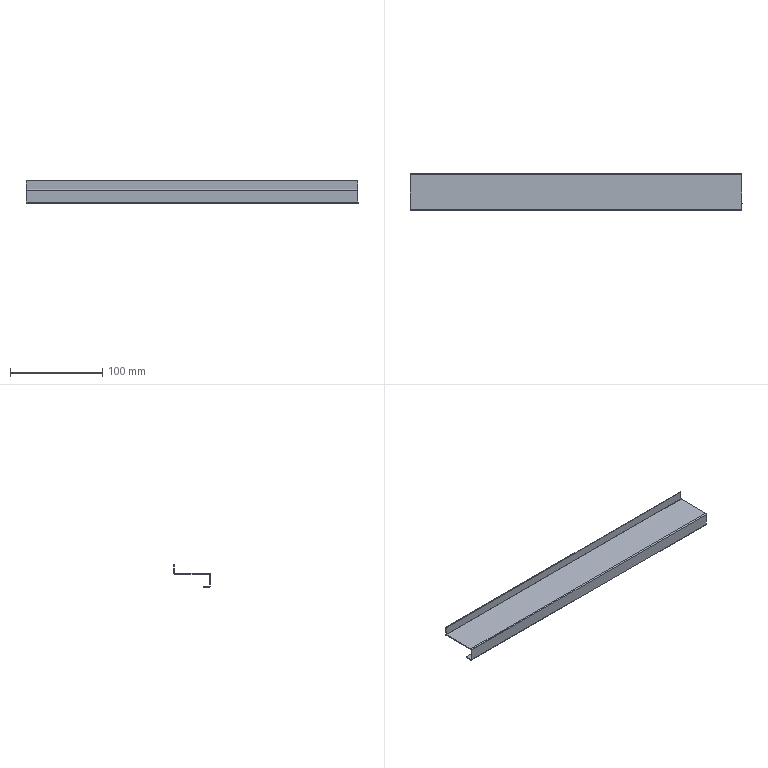Component | SolidWorks | MainBodyWeldment-1_UpperBeam-1 | 1 solid | 30 faces | box 360 x 40 x 24 mm | volume 24922 mm3 | plane 24 | cylinder 6 | commonest cylinder face diameters 0.2 x3 2.2 x3 | material SPCC
STEP:
#1=COLOUR_RGB('',0.7922,0.8196,0.9333);
#2=FILL_AREA_STYLE_COLOUR('',#1);
#3=FILL_AREA_STYLE('',(#2));
#4=SURFACE_STYLE_FILL_AREA(#3);
#5=SURFACE_SIDE_STYLE('',(#4));
#6=SURFACE_STYLE_USAGE(.BOTH.,#5);
#7=PRESENTATION_STYLE_ASSIGNMENT((#6));
#8=CARTESIAN_POINT('',(-7.236,13.105,9.799));
#9=VERTEX_POINT('',#8);
#10=CARTESIAN_POINT('',(-7.236,13.105,9.295));
#11=VERTEX_POINT('',#10);
#12=CARTESIAN_POINT('',(-7.236,13.105,9.843));
#13=DIRECTION('',(0.,0.,-1.));
#14=VECTOR('',#13,39.37);
#15=LINE('',#12,#14);
#16=EDGE_CURVE('',#9,#11,#15,.T.);
#17=ORIENTED_EDGE('',*,*,#16,.T.);
#18=CARTESIAN_POINT('',(-7.236,13.066,9.295));
#19=VERTEX_POINT('',#18);
#20=CARTESIAN_POINT('',(-7.236,13.105,9.295));
#21=DIRECTION('',(-0.,-1.,0.));
#22=VECTOR('',#21,39.37);
#23=LINE('',#20,#22);
#24=EDGE_CURVE('',#11,#19,#23,.T.);
#25=ORIENTED_EDGE('',*,*,#24,.T.);
#26=CARTESIAN_POINT('',(-7.236,13.066,9.799));
#27=VERTEX_POINT('',#26);
#28=CARTESIAN_POINT('',(-7.236,13.066,9.843));
#29=DIRECTION('',(0.,0.,-1.));
#30=VECTOR('',#29,39.37);
#31=LINE('',#28,#30);
#32=EDGE_CURVE('',#27,#19,#31,.T.);
#33=ORIENTED_EDGE('',*,*,#32,.F.);
#34=CARTESIAN_POINT('',(-7.236,13.066,9.799));
#35=DIRECTION('',(0.,1.,0.));
#36=VECTOR('',#35,39.37);
#37=LINE('',#34,#36);
#38=EDGE_CURVE('',#27,#9,#37,.T.);
#39=ORIENTED_EDGE('',*,*,#38,.T.);
#40=EDGE_LOOP('',(#17,#25,#33,#39));
#41=FACE_OUTER_BOUND('',#40,.T.);
#42=CARTESIAN_POINT('',(-7.236,13.109,9.803));
#43=DIRECTION('',(-1.,0.,0.));
#44=DIRECTION('',(0.,0.,1.));
#45=AXIS2_PLACEMENT_3D('',#42,#43,#44);
#46=PLANE('',#45);
#47=ADVANCED_FACE('',(#41),#46,.T.);
#48=CARTESIAN_POINT('',(6.938,13.066,9.295));
#49=VERTEX_POINT('',#48);
#50=CARTESIAN_POINT('',(-7.236,13.066,9.295));
#51=DIRECTION('',(1.,0.,0.));
#52=VECTOR('',#51,39.37);
#53=LINE('',#50,#52);
#54=EDGE_CURVE('',#19,#49,#53,.T.);
#55=ORIENTED_EDGE('',*,*,#54,.T.);
#56=CARTESIAN_POINT('',(6.938,13.066,9.799));
#57=VERTEX_POINT('',#56);
#58=CARTESIAN_POINT('',(6.938,13.066,9.843));
#59=DIRECTION('',(0.,0.,-1.));
#60=VECTOR('',#59,39.37);
#61=LINE('',#58,#60);
#62=EDGE_CURVE('',#57,#49,#61,.T.);
#63=ORIENTED_EDGE('',*,*,#62,.F.);
#64=CARTESIAN_POINT('',(6.938,13.066,9.799));
#65=DIRECTION('',(-1.,0.,0.));
#66=VECTOR('',#65,39.37);
#67=LINE('',#64,#66);
#68=EDGE_CURVE('',#57,#27,#67,.T.);
#69=ORIENTED_EDGE('',*,*,#68,.T.);
#70=ORIENTED_EDGE('',*,*,#32,.T.);
#71=EDGE_LOOP('',(#55,#63,#69,#70));
#72=FACE_OUTER_BOUND('',#71,.T.);
#73=CARTESIAN_POINT('',(6.938,13.066,9.843));
#74=DIRECTION('',(0.,1.,0.));
#75=DIRECTION('',(0.,0.,1.));
#76=AXIS2_PLACEMENT_3D('',#73,#74,#75);
#77=PLANE('',#76);
#78=ADVANCED_FACE('',(#72),#77,.F.);
#79=CARTESIAN_POINT('',(6.938,13.105,9.799));
#80=VERTEX_POINT('',#79);
#81=CARTESIAN_POINT('',(6.938,13.105,9.295));
#82=VERTEX_POINT('',#81);
#83=CARTESIAN_POINT('',(6.938,13.105,9.843));
#84=DIRECTION('',(0.,0.,-1.));
#85=VECTOR('',#84,39.37);
#86=LINE('',#83,#85);
#87=EDGE_CURVE('',#80,#82,#86,.T.);
#88=ORIENTED_EDGE('',*,*,#87,.T.);
#89=CARTESIAN_POINT('',(-7.236,13.105,9.295));
#90=DIRECTION('',(1.,0.,0.));
#91=VECTOR('',#90,39.37);
#92=LINE('',#89,#91);
#93=EDGE_CURVE('',#11,#82,#92,.T.);
#94=ORIENTED_EDGE('',*,*,#93,.F.);
#95=ORIENTED_EDGE('',*,*,#16,.F.);
#96=CARTESIAN_POINT('',(6.938,13.105,9.799));
#97=DIRECTION('',(-1.,0.,0.));
#98=VECTOR('',#97,39.37);
#99=LINE('',#96,#98);
#100=EDGE_CURVE('',#80,#9,#99,.T.);
#101=ORIENTED_EDGE('',*,*,#100,.F.);
#102=EDGE_LOOP('',(#88,#94,#95,#101));
#103=FACE_OUTER_BOUND('',#102,.T.);
#104=CARTESIAN_POINT('',(6.938,13.105,9.843));
#105=DIRECTION('',(0.,1.,0.));
#106=DIRECTION('',(0.,0.,1.));
#107=AXIS2_PLACEMENT_3D('',#104,#105,#106);
#108=PLANE('',#107);
#109=ADVANCED_FACE('',(#103),#108,.T.);
#110=CARTESIAN_POINT('',(6.938,13.109,9.843));
#111=VERTEX_POINT('',#110);
#112=CARTESIAN_POINT('',(6.938,13.109,9.803));
#113=VERTEX_POINT('',#112);
#114=CARTESIAN_POINT('',(6.938,13.109,9.843));
#115=DIRECTION('',(0.,0.,-1.));
#116=VECTOR('',#115,39.37);
#117=LINE('',#114,#116);
#118=EDGE_CURVE('',#111,#113,#117,.T.);
#119=ORIENTED_EDGE('',*,*,#118,.F.);
#120=CARTESIAN_POINT('',(6.938,13.109,9.799));
#121=DIRECTION('',(1.,0.,0.));
#122=DIRECTION('',(0.,0.,-1.));
#123=AXIS2_PLACEMENT_3D('',#120,#121,#122);
#124=CIRCLE('',#123,0.04331);
#125=EDGE_CURVE('',#111,#57,#124,.T.);
#126=ORIENTED_EDGE('',*,*,#125,.T.);
#127=CARTESIAN_POINT('',(6.938,13.105,9.799));
#128=DIRECTION('',(0.,-1.,0.));
#129=VECTOR('',#128,39.37);
#130=LINE('',#127,#129);
#131=EDGE_CURVE('',#80,#57,#130,.T.);
#132=ORIENTED_EDGE('',*,*,#131,.F.);
#133=CARTESIAN_POINT('',(6.938,13.109,9.799));
#134=DIRECTION('',(1.,0.,0.));
#135=DIRECTION('',(0.,0.,-1.));
#136=AXIS2_PLACEMENT_3D('',#133,#134,#135);
#137=CIRCLE('',#136,0.003937);
#138=EDGE_CURVE('',#113,#80,#137,.T.);
#139=ORIENTED_EDGE('',*,*,#138,.F.);
#140=EDGE_LOOP('',(#119,#126,#132,#139));
#141=FACE_OUTER_BOUND('',#140,.T.);
#142=CARTESIAN_POINT('',(6.938,13.109,9.843));
#143=DIRECTION('',(1.,0.,0.));
#144=DIRECTION('',(0.,0.,-1.));
#145=AXIS2_PLACEMENT_3D('',#142,#143,#144);
#146=PLANE('',#145);
#147=ADVANCED_FACE('',(#141),#146,.T.);
#148=CARTESIAN_POINT('',(6.938,14.597,9.843));
#149=VERTEX_POINT('',#148);
#150=CARTESIAN_POINT('',(6.938,13.066,9.843));
#151=DIRECTION('',(0.,-1.,0.));
#152=VECTOR('',#151,39.37);
#153=LINE('',#150,#152);
#154=EDGE_CURVE('',#149,#111,#153,.T.);
#155=ORIENTED_EDGE('',*,*,#154,.T.);
#156=ORIENTED_EDGE('',*,*,#118,.T.);
#157=CARTESIAN_POINT('',(6.938,14.597,9.803));
#158=VERTEX_POINT('',#157);
#159=CARTESIAN_POINT('',(6.938,13.066,9.803));
#160=DIRECTION('',(0.,-1.,0.));
#161=VECTOR('',#160,39.37);
#162=LINE('',#159,#161);
#163=EDGE_CURVE('',#158,#113,#162,.T.);
#164=ORIENTED_EDGE('',*,*,#163,.F.);
#165=CARTESIAN_POINT('',(6.938,14.597,9.803));
#166=DIRECTION('',(0.,0.,1.));
#167=VECTOR('',#166,39.37);
#168=LINE('',#165,#167);
#169=EDGE_CURVE('',#158,#149,#168,.T.);
#170=ORIENTED_EDGE('',*,*,#169,.T.);
#171=EDGE_LOOP('',(#155,#156,#164,#170));
#172=FACE_OUTER_BOUND('',#171,.T.);
#173=CARTESIAN_POINT('',(6.938,13.105,9.799));
#174=DIRECTION('',(1.,0.,0.));
#175=DIRECTION('',(0.,0.,-1.));
#176=AXIS2_PLACEMENT_3D('',#173,#174,#175);
#177=PLANE('',#176);
#178=ADVANCED_FACE('',(#172),#177,.T.);
#179=ORIENTED_EDGE('',*,*,#38,.F.);
#180=CARTESIAN_POINT('',(-7.236,13.109,9.843));
#181=VERTEX_POINT('',#180);
#182=CARTESIAN_POINT('',(-7.236,13.109,9.799));
#183=DIRECTION('',(1.,0.,0.));
#184=DIRECTION('',(0.,0.,-1.));
#185=AXIS2_PLACEMENT_3D('',#182,#183,#184);
#186=CIRCLE('',#185,0.04331);
#187=EDGE_CURVE('',#181,#27,#186,.T.);
#188=ORIENTED_EDGE('',*,*,#187,.F.);
#189=CARTESIAN_POINT('',(-7.236,13.109,9.803));
#190=VERTEX_POINT('',#189);
#191=CARTESIAN_POINT('',(-7.236,13.109,9.803));
#192=DIRECTION('',(0.,0.,1.));
#193=VECTOR('',#192,39.37);
#194=LINE('',#191,#193);
#195=EDGE_CURVE('',#190,#181,#194,.T.);
#196=ORIENTED_EDGE('',*,*,#195,.F.);
#197=CARTESIAN_POINT('',(-7.236,13.109,9.799));
#198=DIRECTION('',(1.,0.,0.));
#199=DIRECTION('',(0.,0.,-1.));
#200=AXIS2_PLACEMENT_3D('',#197,#198,#199);
#201=CIRCLE('',#200,0.003937);
#202=EDGE_CURVE('',#190,#9,#201,.T.);
#203=ORIENTED_EDGE('',*,*,#202,.T.);
#204=EDGE_LOOP('',(#179,#188,#196,#203));
#205=FACE_OUTER_BOUND('',#204,.T.);
#206=CARTESIAN_POINT('',(-7.236,13.066,9.799));
#207=DIRECTION('',(-1.,0.,0.));
#208=DIRECTION('',(0.,0.,1.));
#209=AXIS2_PLACEMENT_3D('',#206,#207,#208);
#210=PLANE('',#209);
#211=ADVANCED_FACE('',(#205),#210,.T.);
#212=CARTESIAN_POINT('',(6.938,14.601,9.847));
#213=VERTEX_POINT('',#212);
#214=CARTESIAN_POINT('',(6.938,14.641,9.847));
#215=VERTEX_POINT('',#214);
#216=CARTESIAN_POINT('',(6.938,14.601,9.847));
#217=DIRECTION('',(0.,1.,-0.));
#218=VECTOR('',#217,39.37);
#219=LINE('',#216,#218);
#220=EDGE_CURVE('',#213,#215,#219,.T.);
#221=ORIENTED_EDGE('',*,*,#220,.F.);
#222=CARTESIAN_POINT('',(6.938,14.597,9.847));
#223=DIRECTION('',(-1.,0.,0.));
#224=DIRECTION('',(0.,0.,1.));
#225=AXIS2_PLACEMENT_3D('',#222,#223,#224);
#226=CIRCLE('',#225,0.003937);
#227=EDGE_CURVE('',#213,#149,#226,.T.);
#228=ORIENTED_EDGE('',*,*,#227,.T.);
#229=ORIENTED_EDGE('',*,*,#169,.F.);
#230=CARTESIAN_POINT('',(6.938,14.597,9.847));
#231=DIRECTION('',(-1.,0.,0.));
#232=DIRECTION('',(0.,0.,-1.));
#233=AXIS2_PLACEMENT_3D('',#230,#231,#232);
#234=CIRCLE('',#233,0.04331);
#235=EDGE_CURVE('',#215,#158,#234,.T.);
#236=ORIENTED_EDGE('',*,*,#235,.F.);
#237=EDGE_LOOP('',(#221,#228,#229,#236));
#238=FACE_OUTER_BOUND('',#237,.T.);
#239=CARTESIAN_POINT('',(6.938,14.601,9.847));
#240=DIRECTION('',(1.,0.,0.));
#241=DIRECTION('',(0.,0.,-1.));
#242=AXIS2_PLACEMENT_3D('',#239,#240,#241);
#243=PLANE('',#242);
#244=ADVANCED_FACE('',(#238),#243,.T.);
#245=CARTESIAN_POINT('',(6.938,14.601,10.197));
#246=VERTEX_POINT('',#245);
#247=CARTESIAN_POINT('',(6.938,14.601,9.843));
#248=DIRECTION('',(0.,0.,-1.));
#249=VECTOR('',#248,39.37);
#250=LINE('',#247,#249);
#251=EDGE_CURVE('',#246,#213,#250,.T.);
#252=ORIENTED_EDGE('',*,*,#251,.T.);
#253=ORIENTED_EDGE('',*,*,#220,.T.);
#254=CARTESIAN_POINT('',(6.938,14.641,10.197));
#255=VERTEX_POINT('',#254);
#256=CARTESIAN_POINT('',(6.938,14.641,9.843));
#257=DIRECTION('',(0.,0.,-1.));
#258=VECTOR('',#257,39.37);
#259=LINE('',#256,#258);
#260=EDGE_CURVE('',#255,#215,#259,.T.);
#261=ORIENTED_EDGE('',*,*,#260,.F.);
#262=CARTESIAN_POINT('',(6.938,14.601,10.197));
#263=DIRECTION('',(0.,1.,0.));
#264=VECTOR('',#263,39.37);
#265=LINE('',#262,#264);
#266=EDGE_CURVE('',#246,#255,#265,.T.);
#267=ORIENTED_EDGE('',*,*,#266,.F.);
#268=EDGE_LOOP('',(#252,#253,#261,#267));
#269=FACE_OUTER_BOUND('',#268,.T.);
#270=CARTESIAN_POINT('',(6.938,14.597,9.803));
#271=DIRECTION('',(1.,0.,0.));
#272=DIRECTION('',(0.,0.,-1.));
#273=AXIS2_PLACEMENT_3D('',#270,#271,#272);
#274=PLANE('',#273);
#275=ADVANCED_FACE('',(#269),#274,.T.);
#276=CARTESIAN_POINT('',(-7.236,14.597,9.843));
#277=VERTEX_POINT('',#276);
#278=CARTESIAN_POINT('',(-7.236,14.597,9.803));
#279=VERTEX_POINT('',#278);
#280=CARTESIAN_POINT('',(-7.236,14.597,9.843));
#281=DIRECTION('',(0.,0.,-1.));
#282=VECTOR('',#281,39.37);
#283=LINE('',#280,#282);
#284=EDGE_CURVE('',#277,#279,#283,.T.);
#285=ORIENTED_EDGE('',*,*,#284,.F.);
#286=CARTESIAN_POINT('',(-7.236,14.601,9.847));
#287=VERTEX_POINT('',#286);
#288=CARTESIAN_POINT('',(-7.236,14.597,9.847));
#289=DIRECTION('',(-1.,0.,0.));
#290=DIRECTION('',(0.,0.,1.));
#291=AXIS2_PLACEMENT_3D('',#288,#289,#290);
#292=CIRCLE('',#291,0.003937);
#293=EDGE_CURVE('',#287,#277,#292,.T.);
#294=ORIENTED_EDGE('',*,*,#293,.F.);
#295=CARTESIAN_POINT('',(-7.236,14.641,9.847));
#296=VERTEX_POINT('',#295);
#297=CARTESIAN_POINT('',(-7.236,14.641,9.847));
#298=DIRECTION('',(0.,-1.,0.));
#299=VECTOR('',#298,39.37);
#300=LINE('',#297,#299);
#301=EDGE_CURVE('',#296,#287,#300,.T.);
#302=ORIENTED_EDGE('',*,*,#301,.F.);
#303=CARTESIAN_POINT('',(-7.236,14.597,9.847));
#304=DIRECTION('',(-1.,0.,0.));
#305=DIRECTION('',(0.,0.,-1.));
#306=AXIS2_PLACEMENT_3D('',#303,#304,#305);
#307=CIRCLE('',#306,0.04331);
#308=EDGE_CURVE('',#296,#279,#307,.T.);
#309=ORIENTED_EDGE('',*,*,#308,.T.);
#310=EDGE_LOOP('',(#285,#294,#302,#309));
#311=FACE_OUTER_BOUND('',#310,.T.);
#312=CARTESIAN_POINT('',(-7.236,14.597,9.843));
#313=DIRECTION('',(-1.,0.,0.));
#314=DIRECTION('',(0.,0.,1.));
#315=AXIS2_PLACEMENT_3D('',#312,#313,#314);
#316=PLANE('',#315);
#317=ADVANCED_FACE('',(#311),#316,.T.);
#318=CARTESIAN_POINT('',(-7.236,13.066,9.843));
#319=DIRECTION('',(0.,-1.,0.));
#320=VECTOR('',#319,39.37);
#321=LINE('',#318,#320);
#322=EDGE_CURVE('',#277,#181,#321,.T.);
#323=ORIENTED_EDGE('',*,*,#322,.F.);
#324=ORIENTED_EDGE('',*,*,#284,.T.);
#325=CARTESIAN_POINT('',(-7.236,13.066,9.803));
#326=DIRECTION('',(0.,-1.,0.));
#327=VECTOR('',#326,39.37);
#328=LINE('',#325,#327);
#329=EDGE_CURVE('',#279,#190,#328,.T.);
#330=ORIENTED_EDGE('',*,*,#329,.T.);
#331=ORIENTED_EDGE('',*,*,#195,.T.);
#332=EDGE_LOOP('',(#323,#324,#330,#331));
#333=FACE_OUTER_BOUND('',#332,.T.);
#334=CARTESIAN_POINT('',(-7.236,14.641,9.847));
#335=DIRECTION('',(-1.,0.,0.));
#336=DIRECTION('',(0.,0.,1.));
#337=AXIS2_PLACEMENT_3D('',#334,#335,#336);
#338=PLANE('',#337);
#339=ADVANCED_FACE('',(#333),#338,.T.);
#340=ORIENTED_EDGE('',*,*,#202,.F.);
#341=CARTESIAN_POINT('',(6.938,13.109,9.803));
#342=DIRECTION('',(-1.,0.,0.));
#343=VECTOR('',#342,39.37);
#344=LINE('',#341,#343);
#345=EDGE_CURVE('',#113,#190,#344,.T.);
#346=ORIENTED_EDGE('',*,*,#345,.F.);
#347=ORIENTED_EDGE('',*,*,#138,.T.);
#348=ORIENTED_EDGE('',*,*,#100,.T.);
#349=EDGE_LOOP('',(#340,#346,#347,#348));
#350=FACE_OUTER_BOUND('',#349,.T.);
#351=CARTESIAN_POINT('',(6.938,13.109,9.799));
#352=DIRECTION('',(-1.,0.,0.));
#353=DIRECTION('',(0.,0.,1.));
#354=AXIS2_PLACEMENT_3D('',#351,#352,#353);
#355=CYLINDRICAL_SURFACE('',#354,0.003937);
#356=ADVANCED_FACE('',(#350),#355,.F.);
#357=ORIENTED_EDGE('',*,*,#329,.F.);
#358=CARTESIAN_POINT('',(6.938,14.597,9.803));
#359=DIRECTION('',(-1.,0.,0.));
#360=VECTOR('',#359,39.37);
#361=LINE('',#358,#360);
#362=EDGE_CURVE('',#158,#279,#361,.T.);
#363=ORIENTED_EDGE('',*,*,#362,.F.);
#364=ORIENTED_EDGE('',*,*,#163,.T.);
#365=ORIENTED_EDGE('',*,*,#345,.T.);
#366=EDGE_LOOP('',(#357,#363,#364,#365));
#367=FACE_OUTER_BOUND('',#366,.T.);
#368=CARTESIAN_POINT('',(6.938,13.066,9.803));
#369=DIRECTION('',(0.,0.,-1.));
#370=DIRECTION('',(-1.,0.,0.));
#371=AXIS2_PLACEMENT_3D('',#368,#369,#370);
#372=PLANE('',#371);
#373=ADVANCED_FACE('',(#367),#372,.T.);
#374=ORIENTED_EDGE('',*,*,#308,.F.);
#375=CARTESIAN_POINT('',(6.938,14.641,9.847));
#376=DIRECTION('',(-1.,0.,0.));
#377=VECTOR('',#376,39.37);
#378=LINE('',#375,#377);
#379=EDGE_CURVE('',#215,#296,#378,.T.);
#380=ORIENTED_EDGE('',*,*,#379,.F.);
#381=ORIENTED_EDGE('',*,*,#235,.T.);
#382=ORIENTED_EDGE('',*,*,#362,.T.);
#383=EDGE_LOOP('',(#374,#380,#381,#382));
#384=FACE_OUTER_BOUND('',#383,.T.);
#385=CARTESIAN_POINT('',(6.938,14.597,9.847));
#386=DIRECTION('',(-1.,0.,0.));
#387=DIRECTION('',(0.,0.,1.));
#388=AXIS2_PLACEMENT_3D('',#385,#386,#387);
#389=CYLINDRICAL_SURFACE('',#388,0.04331);
#390=ADVANCED_FACE('',(#384),#389,.T.);
#391=CARTESIAN_POINT('',(-7.236,14.641,10.197));
#392=VERTEX_POINT('',#391);
#393=CARTESIAN_POINT('',(-7.236,14.641,9.843));
#394=DIRECTION('',(0.,0.,-1.));
#395=VECTOR('',#394,39.37);
#396=LINE('',#393,#395);
#397=EDGE_CURVE('',#392,#296,#396,.T.);
#398=ORIENTED_EDGE('',*,*,#397,.F.);
#399=CARTESIAN_POINT('',(6.938,14.641,10.197));
#400=DIRECTION('',(-1.,0.,0.));
#401=VECTOR('',#400,39.37);
#402=LINE('',#399,#401);
#403=EDGE_CURVE('',#255,#392,#402,.T.);
#404=ORIENTED_EDGE('',*,*,#403,.F.);
#405=ORIENTED_EDGE('',*,*,#260,.T.);
#406=ORIENTED_EDGE('',*,*,#379,.T.);
#407=EDGE_LOOP('',(#398,#404,#405,#406));
#408=FACE_OUTER_BOUND('',#407,.T.);
#409=CARTESIAN_POINT('',(6.938,14.641,9.843));
#410=DIRECTION('',(0.,1.,0.));
#411=DIRECTION('',(0.,0.,1.));
#412=AXIS2_PLACEMENT_3D('',#409,#410,#411);
#413=PLANE('',#412);
#414=ADVANCED_FACE('',(#408),#413,.T.);
#415=CARTESIAN_POINT('',(-7.236,14.601,10.197));
#416=VERTEX_POINT('',#415);
#417=CARTESIAN_POINT('',(-7.236,14.601,10.197));
#418=DIRECTION('',(0.,1.,0.));
#419=VECTOR('',#418,39.37);
#420=LINE('',#417,#419);
#421=EDGE_CURVE('',#416,#392,#420,.T.);
#422=ORIENTED_EDGE('',*,*,#421,.F.);
#423=CARTESIAN_POINT('',(6.938,14.601,10.197));
#424=DIRECTION('',(-1.,0.,0.));
#425=VECTOR('',#424,39.37);
#426=LINE('',#423,#425);
#427=EDGE_CURVE('',#246,#416,#426,.T.);
#428=ORIENTED_EDGE('',*,*,#427,.F.);
#429=ORIENTED_EDGE('',*,*,#266,.T.);
#430=ORIENTED_EDGE('',*,*,#403,.T.);
#431=EDGE_LOOP('',(#422,#428,#429,#430));
#432=FACE_OUTER_BOUND('',#431,.T.);
#433=CARTESIAN_POINT('',(6.938,14.601,10.197));
#434=DIRECTION('',(0.,0.,1.));
#435=DIRECTION('',(1.,0.,0.));
#436=AXIS2_PLACEMENT_3D('',#433,#434,#435);
#437=PLANE('',#436);
#438=ADVANCED_FACE('',(#432),#437,.T.);
#439=CARTESIAN_POINT('',(-7.236,14.601,9.843));
#440=DIRECTION('',(0.,0.,-1.));
#441=VECTOR('',#440,39.37);
#442=LINE('',#439,#441);
#443=EDGE_CURVE('',#416,#287,#442,.T.);
#444=ORIENTED_EDGE('',*,*,#443,.T.);
#445=CARTESIAN_POINT('',(6.938,14.601,9.847));
#446=DIRECTION('',(-1.,0.,0.));
#447=VECTOR('',#446,39.37);
#448=LINE('',#445,#447);
#449=EDGE_CURVE('',#213,#287,#448,.T.);
#450=ORIENTED_EDGE('',*,*,#449,.F.);
#451=ORIENTED_EDGE('',*,*,#251,.F.);
#452=ORIENTED_EDGE('',*,*,#427,.T.);
#453=EDGE_LOOP('',(#444,#450,#451,#452));
#454=FACE_OUTER_BOUND('',#453,.T.);
#455=CARTESIAN_POINT('',(6.938,14.601,9.843));
#456=DIRECTION('',(0.,1.,0.));
#457=DIRECTION('',(0.,0.,1.));
#458=AXIS2_PLACEMENT_3D('',#455,#456,#457);
#459=PLANE('',#458);
#460=ADVANCED_FACE('',(#454),#459,.F.);
#461=ORIENTED_EDGE('',*,*,#293,.T.);
#462=CARTESIAN_POINT('',(6.938,14.597,9.843));
#463=DIRECTION('',(-1.,0.,0.));
#464=VECTOR('',#463,39.37);
#465=LINE('',#462,#464);
#466=EDGE_CURVE('',#149,#277,#465,.T.);
#467=ORIENTED_EDGE('',*,*,#466,.F.);
#468=ORIENTED_EDGE('',*,*,#227,.F.);
#469=ORIENTED_EDGE('',*,*,#449,.T.);
#470=EDGE_LOOP('',(#461,#467,#468,#469));
#471=FACE_OUTER_BOUND('',#470,.T.);
#472=CARTESIAN_POINT('',(6.938,14.597,9.847));
#473=DIRECTION('',(-1.,0.,0.));
#474=DIRECTION('',(0.,0.,1.));
#475=AXIS2_PLACEMENT_3D('',#472,#473,#474);
#476=CYLINDRICAL_SURFACE('',#475,0.003937);
#477=ADVANCED_FACE('',(#471),#476,.F.);
#478=ORIENTED_EDGE('',*,*,#322,.T.);
#479=CARTESIAN_POINT('',(6.938,13.109,9.843));
#480=DIRECTION('',(-1.,0.,0.));
#481=VECTOR('',#480,39.37);
#482=LINE('',#479,#481);
#483=EDGE_CURVE('',#111,#181,#482,.T.);
#484=ORIENTED_EDGE('',*,*,#483,.F.);
#485=ORIENTED_EDGE('',*,*,#154,.F.);
#486=ORIENTED_EDGE('',*,*,#466,.T.);
#487=EDGE_LOOP('',(#478,#484,#485,#486));
#488=FACE_OUTER_BOUND('',#487,.T.);
#489=CARTESIAN_POINT('',(6.938,13.066,9.843));
#490=DIRECTION('',(0.,0.,-1.));
#491=DIRECTION('',(-1.,0.,0.));
#492=AXIS2_PLACEMENT_3D('',#489,#490,#491);
#493=PLANE('',#492);
#494=ADVANCED_FACE('',(#488),#493,.F.);
#495=ORIENTED_EDGE('',*,*,#187,.T.);
#496=ORIENTED_EDGE('',*,*,#68,.F.);
#497=ORIENTED_EDGE('',*,*,#125,.F.);
#498=ORIENTED_EDGE('',*,*,#483,.T.);
#499=EDGE_LOOP('',(#495,#496,#497,#498));
#500=FACE_OUTER_BOUND('',#499,.T.);
#501=CARTESIAN_POINT('',(6.938,13.109,9.799));
#502=DIRECTION('',(-1.,0.,0.));
#503=DIRECTION('',(0.,0.,1.));
#504=AXIS2_PLACEMENT_3D('',#501,#502,#503);
#505=CYLINDRICAL_SURFACE('',#504,0.04331);
#506=ADVANCED_FACE('',(#500),#505,.T.);
#507=CARTESIAN_POINT('',(6.938,13.105,9.295));
#508=DIRECTION('',(0.,-1.,0.));
#509=VECTOR('',#508,39.37);
#510=LINE('',#507,#509);
#511=EDGE_CURVE('',#82,#49,#510,.T.);
#512=ORIENTED_EDGE('',*,*,#511,.F.);
#513=ORIENTED_EDGE('',*,*,#87,.F.);
#514=ORIENTED_EDGE('',*,*,#131,.T.);
#515=ORIENTED_EDGE('',*,*,#62,.T.);
#516=EDGE_LOOP('',(#512,#513,#514,#515));
#517=FACE_OUTER_BOUND('',#516,.T.);
#518=CARTESIAN_POINT('',(6.938,13.109,9.799));
#519=DIRECTION('',(1.,0.,0.));
#520=DIRECTION('',(0.,0.,-1.));
#521=AXIS2_PLACEMENT_3D('',#518,#519,#520);
#522=PLANE('',#521);
#523=ADVANCED_FACE('',(#517),#522,.T.);
#524=ORIENTED_EDGE('',*,*,#397,.T.);
#525=ORIENTED_EDGE('',*,*,#301,.T.);
#526=ORIENTED_EDGE('',*,*,#443,.F.);
#527=ORIENTED_EDGE('',*,*,#421,.T.);
#528=EDGE_LOOP('',(#524,#525,#526,#527));
#529=FACE_OUTER_BOUND('',#528,.T.);
#530=CARTESIAN_POINT('',(-7.236,13.109,9.799));
#531=DIRECTION('',(1.,0.,0.));
#532=DIRECTION('',(0.,0.,-1.));
#533=AXIS2_PLACEMENT_3D('',#530,#531,#532);
#534=PLANE('',#533);
#535=ADVANCED_FACE('',(#529),#534,.F.);
#536=CARTESIAN_POINT('',(6.938,13.109,9.291));
#537=VERTEX_POINT('',#536);
#538=CARTESIAN_POINT('',(6.938,13.109,9.252));
#539=VERTEX_POINT('',#538);
#540=CARTESIAN_POINT('',(6.938,13.109,9.252));
#541=DIRECTION('',(0.,0.,-1.));
#542=VECTOR('',#541,39.37);
#543=LINE('',#540,#542);
#544=EDGE_CURVE('',#537,#539,#543,.T.);
#545=ORIENTED_EDGE('',*,*,#544,.F.);
#546=CARTESIAN_POINT('',(6.938,13.109,9.295));
#547=DIRECTION('',(1.,0.,0.));
#548=DIRECTION('',(0.,0.,1.));
#549=AXIS2_PLACEMENT_3D('',#546,#547,#548);
#550=CIRCLE('',#549,0.003937);
#551=EDGE_CURVE('',#82,#537,#550,.T.);
#552=ORIENTED_EDGE('',*,*,#551,.F.);
#553=ORIENTED_EDGE('',*,*,#511,.T.);
#554=CARTESIAN_POINT('',(6.938,13.109,9.295));
#555=DIRECTION('',(1.,0.,0.));
#556=DIRECTION('',(0.,0.,1.));
#557=AXIS2_PLACEMENT_3D('',#554,#555,#556);
#558=CIRCLE('',#557,0.04331);
#559=EDGE_CURVE('',#49,#539,#558,.T.);
#560=ORIENTED_EDGE('',*,*,#559,.T.);
#561=EDGE_LOOP('',(#545,#552,#553,#560));
#562=FACE_OUTER_BOUND('',#561,.T.);
#563=CARTESIAN_POINT('',(6.938,13.109,9.295));
#564=DIRECTION('',(1.,0.,0.));
#565=DIRECTION('',(0.,0.,-1.));
#566=AXIS2_PLACEMENT_3D('',#563,#564,#565);
#567=PLANE('',#566);
#568=ADVANCED_FACE('',(#562),#567,.T.);
#569=CARTESIAN_POINT('',(-7.236,13.109,9.291));
#570=VERTEX_POINT('',#569);
#571=CARTESIAN_POINT('',(-7.236,13.109,9.295));
#572=DIRECTION('',(-1.,0.,0.));
#573=DIRECTION('',(0.,0.,1.));
#574=AXIS2_PLACEMENT_3D('',#571,#572,#573);
#575=CIRCLE('',#574,0.003937);
#576=EDGE_CURVE('',#570,#11,#575,.T.);
#577=ORIENTED_EDGE('',*,*,#576,.F.);
#578=CARTESIAN_POINT('',(-7.236,13.109,9.252));
#579=VERTEX_POINT('',#578);
#580=CARTESIAN_POINT('',(-7.236,13.109,9.291));
#581=DIRECTION('',(0.,0.,-1.));
#582=VECTOR('',#581,39.37);
#583=LINE('',#580,#582);
#584=EDGE_CURVE('',#570,#579,#583,.T.);
#585=ORIENTED_EDGE('',*,*,#584,.T.);
#586=CARTESIAN_POINT('',(-7.236,13.109,9.295));
#587=DIRECTION('',(-1.,0.,0.));
#588=DIRECTION('',(0.,0.,1.));
#589=AXIS2_PLACEMENT_3D('',#586,#587,#588);
#590=CIRCLE('',#589,0.04331);
#591=EDGE_CURVE('',#579,#19,#590,.T.);
#592=ORIENTED_EDGE('',*,*,#591,.T.);
#593=ORIENTED_EDGE('',*,*,#24,.F.);
#594=EDGE_LOOP('',(#577,#585,#592,#593));
#595=FACE_OUTER_BOUND('',#594,.T.);
#596=CARTESIAN_POINT('',(-7.236,13.109,9.295));
#597=DIRECTION('',(1.,0.,0.));
#598=DIRECTION('',(0.,0.,-1.));
#599=AXIS2_PLACEMENT_3D('',#596,#597,#598);
#600=PLANE('',#599);
#601=ADVANCED_FACE('',(#595),#600,.F.);
#602=ORIENTED_EDGE('',*,*,#54,.F.);
#603=ORIENTED_EDGE('',*,*,#591,.F.);
#604=CARTESIAN_POINT('',(-7.236,13.109,9.252));
#605=DIRECTION('',(-1.,0.,0.));
#606=VECTOR('',#605,39.37);
#607=LINE('',#604,#606);
#608=EDGE_CURVE('',#539,#579,#607,.T.);
#609=ORIENTED_EDGE('',*,*,#608,.F.);
#610=ORIENTED_EDGE('',*,*,#559,.F.);
#611=EDGE_LOOP('',(#602,#603,#609,#610));
#612=FACE_OUTER_BOUND('',#611,.T.);
#613=CARTESIAN_POINT('',(-7.236,13.109,9.295));
#614=DIRECTION('',(-1.,0.,0.));
#615=DIRECTION('',(0.,0.,-1.));
#616=AXIS2_PLACEMENT_3D('',#613,#614,#615);
#617=CYLINDRICAL_SURFACE('',#616,0.04331);
#618=ADVANCED_FACE('',(#612),#617,.T.);
#619=ORIENTED_EDGE('',*,*,#93,.T.);
#620=ORIENTED_EDGE('',*,*,#551,.T.);
#621=CARTESIAN_POINT('',(6.938,13.109,9.291));
#622=DIRECTION('',(-1.,0.,0.));
#623=VECTOR('',#622,39.37);
#624=LINE('',#621,#623);
#625=EDGE_CURVE('',#537,#570,#624,.T.);
#626=ORIENTED_EDGE('',*,*,#625,.T.);
#627=ORIENTED_EDGE('',*,*,#576,.T.);
#628=EDGE_LOOP('',(#619,#620,#626,#627));
#629=FACE_OUTER_BOUND('',#628,.T.);
#630=CARTESIAN_POINT('',(-7.236,13.109,9.295));
#631=DIRECTION('',(-1.,0.,0.));
#632=DIRECTION('',(0.,0.,-1.));
#633=AXIS2_PLACEMENT_3D('',#630,#631,#632);
#634=CYLINDRICAL_SURFACE('',#633,0.003937);
#635=ADVANCED_FACE('',(#629),#634,.F.);
#636=CARTESIAN_POINT('',(-7.236,13.381,9.252));
#637=VERTEX_POINT('',#636);
#638=CARTESIAN_POINT('',(-7.236,13.105,9.252));
#639=DIRECTION('',(-0.,-1.,0.));
#640=VECTOR('',#639,39.37);
#641=LINE('',#638,#640);
#642=EDGE_CURVE('',#637,#579,#641,.T.);
#643=ORIENTED_EDGE('',*,*,#642,.T.);
#644=ORIENTED_EDGE('',*,*,#584,.F.);
#645=CARTESIAN_POINT('',(-7.236,13.381,9.291));
#646=VERTEX_POINT('',#645);
#647=CARTESIAN_POINT('',(-7.236,13.066,9.291));
#648=DIRECTION('',(-0.,-1.,0.));
#649=VECTOR('',#648,39.37);
#650=LINE('',#647,#649);
#651=EDGE_CURVE('',#646,#570,#650,.T.);
#652=ORIENTED_EDGE('',*,*,#651,.F.);
#653=CARTESIAN_POINT('',(-7.236,13.381,9.252));
#654=DIRECTION('',(0.,0.,1.));
#655=VECTOR('',#654,39.37);
#656=LINE('',#653,#655);
#657=EDGE_CURVE('',#637,#646,#656,.T.);
#658=ORIENTED_EDGE('',*,*,#657,.F.);
#659=EDGE_LOOP('',(#643,#644,#652,#658));
#660=FACE_OUTER_BOUND('',#659,.T.);
#661=CARTESIAN_POINT('',(-7.236,13.105,9.252));
#662=DIRECTION('',(-1.,0.,0.));
#663=DIRECTION('',(-0.,-1.,0.));
#664=AXIS2_PLACEMENT_3D('',#661,#662,#663);
#665=PLANE('',#664);
#666=ADVANCED_FACE('',(#660),#665,.T.);
#667=CARTESIAN_POINT('',(6.938,13.381,9.291));
#668=VERTEX_POINT('',#667);
#669=CARTESIAN_POINT('',(6.938,13.066,9.291));
#670=DIRECTION('',(0.,1.,0.));
#671=VECTOR('',#670,39.37);
#672=LINE('',#669,#671);
#673=EDGE_CURVE('',#537,#668,#672,.T.);
#674=ORIENTED_EDGE('',*,*,#673,.F.);
#675=ORIENTED_EDGE('',*,*,#544,.T.);
#676=CARTESIAN_POINT('',(6.938,13.381,9.252));
#677=VERTEX_POINT('',#676);
#678=CARTESIAN_POINT('',(6.938,13.381,9.252));
#679=DIRECTION('',(0.,1.,0.));
#680=VECTOR('',#679,39.37);
#681=LINE('',#678,#680);
#682=EDGE_CURVE('',#539,#677,#681,.T.);
#683=ORIENTED_EDGE('',*,*,#682,.T.);
#684=CARTESIAN_POINT('',(6.938,13.381,9.252));
#685=DIRECTION('',(0.,0.,1.));
#686=VECTOR('',#685,39.37);
#687=LINE('',#684,#686);
#688=EDGE_CURVE('',#677,#668,#687,.T.);
#689=ORIENTED_EDGE('',*,*,#688,.T.);
#690=EDGE_LOOP('',(#674,#675,#683,#689));
#691=FACE_OUTER_BOUND('',#690,.T.);
#692=CARTESIAN_POINT('',(6.938,13.381,9.252));
#693=DIRECTION('',(1.,-0.,0.));
#694=DIRECTION('',(0.,1.,0.));
#695=AXIS2_PLACEMENT_3D('',#692,#693,#694);
#696=PLANE('',#695);
#697=ADVANCED_FACE('',(#691),#696,.T.);
#698=ORIENTED_EDGE('',*,*,#682,.F.);
#699=ORIENTED_EDGE('',*,*,#608,.T.);
#700=ORIENTED_EDGE('',*,*,#642,.F.);
#701=CARTESIAN_POINT('',(-7.236,13.381,9.252));
#702=DIRECTION('',(-1.,0.,0.));
#703=VECTOR('',#702,39.37);
#704=LINE('',#701,#703);
#705=EDGE_CURVE('',#677,#637,#704,.T.);
#706=ORIENTED_EDGE('',*,*,#705,.F.);
#707=EDGE_LOOP('',(#698,#699,#700,#706));
#708=FACE_OUTER_BOUND('',#707,.T.);
#709=CARTESIAN_POINT('',(-7.236,13.066,9.252));
#710=DIRECTION('',(0.,0.,-1.));
#711=DIRECTION('',(-1.,0.,0.));
#712=AXIS2_PLACEMENT_3D('',#709,#710,#711);
#713=PLANE('',#712);
#714=ADVANCED_FACE('',(#708),#713,.T.);
#715=ORIENTED_EDGE('',*,*,#625,.F.);
#716=ORIENTED_EDGE('',*,*,#673,.T.);
#717=CARTESIAN_POINT('',(-7.236,13.381,9.291));
#718=DIRECTION('',(-1.,0.,0.));
#719=VECTOR('',#718,39.37);
#720=LINE('',#717,#719);
#721=EDGE_CURVE('',#668,#646,#720,.T.);
#722=ORIENTED_EDGE('',*,*,#721,.T.);
#723=ORIENTED_EDGE('',*,*,#651,.T.);
#724=EDGE_LOOP('',(#715,#716,#722,#723));
#725=FACE_OUTER_BOUND('',#724,.T.);
#726=CARTESIAN_POINT('',(-7.236,13.066,9.291));
#727=DIRECTION('',(0.,0.,-1.));
#728=DIRECTION('',(-1.,0.,0.));
#729=AXIS2_PLACEMENT_3D('',#726,#727,#728);
#730=PLANE('',#729);
#731=ADVANCED_FACE('',(#725),#730,.F.);
#732=ORIENTED_EDGE('',*,*,#721,.F.);
#733=ORIENTED_EDGE('',*,*,#688,.F.);
#734=ORIENTED_EDGE('',*,*,#705,.T.);
#735=ORIENTED_EDGE('',*,*,#657,.T.);
#736=EDGE_LOOP('',(#732,#733,#734,#735));
#737=FACE_OUTER_BOUND('',#736,.T.);
#738=CARTESIAN_POINT('',(-7.236,13.381,9.252));
#739=DIRECTION('',(0.,1.,0.));
#740=DIRECTION('',(0.,0.,1.));
#741=AXIS2_PLACEMENT_3D('',#738,#739,#740);
#742=PLANE('',#741);
#743=ADVANCED_FACE('',(#737),#742,.T.);
#744=CLOSED_SHELL('',(#47,#78,#109,#147,#178,#211,#244,#275,#317,#339,#356,#373,#390,#414,#438,#460,#477,#494,#506,#523,#535,#568,#601,#618,#635,#666,#697,#714,#731,#743));
#745=MANIFOLD_SOLID_BREP('',#744);
#746=STYLED_ITEM('',(#7),#745);
#747=(LENGTH_UNIT()NAMED_UNIT(*)SI_UNIT($,.METRE.));
#748=LENGTH_MEASURE_WITH_UNIT(LENGTH_MEASURE(0.0254),#747);
#749=DIMENSIONAL_EXPONENTS(1.,0.,0.,0.,0.,0.,0.);
#750=(CONVERSION_BASED_UNIT('',#748)LENGTH_UNIT()NAMED_UNIT(#749));
#751=UNCERTAINTY_MEASURE_WITH_UNIT(LENGTH_MEASURE(0.00001),#750,'','');
#752=(NAMED_UNIT(*)PLANE_ANGLE_UNIT()SI_UNIT($,.RADIAN.));
#753=(NAMED_UNIT(*)SI_UNIT($,.STERADIAN.)SOLID_ANGLE_UNIT());
#754=(GEOMETRIC_REPRESENTATION_CONTEXT(3)GLOBAL_UNCERTAINTY_ASSIGNED_CONTEXT((#751))GLOBAL_UNIT_ASSIGNED_CONTEXT((#750,#752,#753))REPRESENTATION_CONTEXT('',''));
#755=MECHANICAL_DESIGN_GEOMETRIC_PRESENTATION_REPRESENTATION('',(#746),#754);
#756=CARTESIAN_POINT('',(0.,0.,0.));
#757=DIRECTION('',(0.,0.,1.));
#758=DIRECTION('',(1.,0.,0.));
#759=AXIS2_PLACEMENT_3D('',#756,#757,#758);
#760=(LENGTH_UNIT()NAMED_UNIT(*)SI_UNIT($,.METRE.));
#761=LENGTH_MEASURE_WITH_UNIT(LENGTH_MEASURE(0.0254),#760);
#762=DIMENSIONAL_EXPONENTS(1.,0.,0.,0.,0.,0.,0.);
#763=(CONVERSION_BASED_UNIT('',#761)LENGTH_UNIT()NAMED_UNIT(#762));
#764=UNCERTAINTY_MEASURE_WITH_UNIT(LENGTH_MEASURE(0.00001),#763,'','');
#765=(NAMED_UNIT(*)PLANE_ANGLE_UNIT()SI_UNIT($,.RADIAN.));
#766=(NAMED_UNIT(*)SI_UNIT($,.STERADIAN.)SOLID_ANGLE_UNIT());
#767=(GEOMETRIC_REPRESENTATION_CONTEXT(3)GLOBAL_UNCERTAINTY_ASSIGNED_CONTEXT((#764))GLOBAL_UNIT_ASSIGNED_CONTEXT((#763,#765,#766))REPRESENTATION_CONTEXT('',''));
#768=ADVANCED_BREP_SHAPE_REPRESENTATION('',(#745,#759),#767);
#769=PRESENTATION_LAYER_ASSIGNMENT('','',(#746));